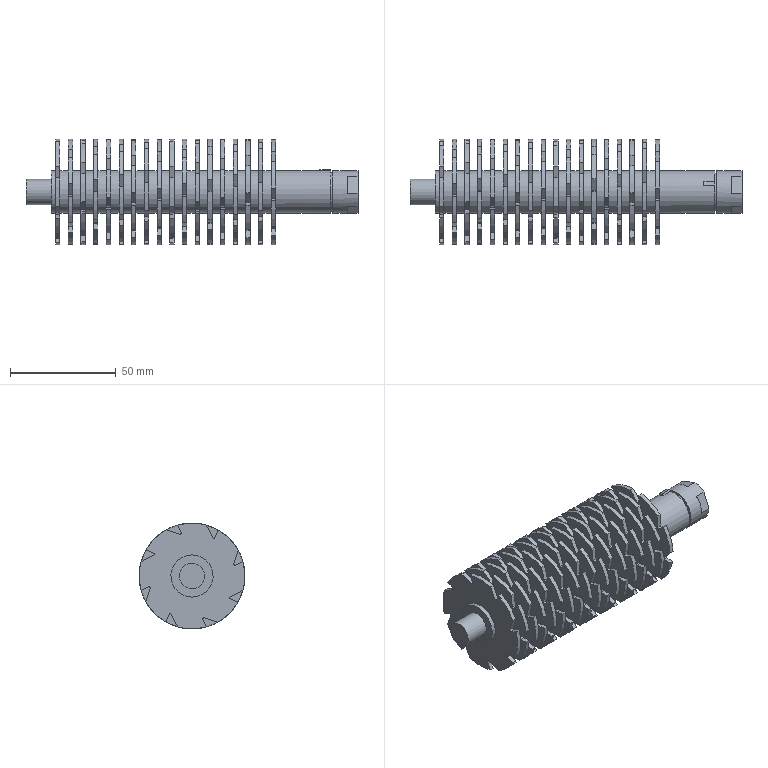Component | NX | SHE_JI-4_2 | 1 solid | 651 faces | volume 101634 mm3 | plane 341 | cylinder 310 | commonest cylinder face diameters 50 x144 1 x144 20 x20 12 x1 18 x1